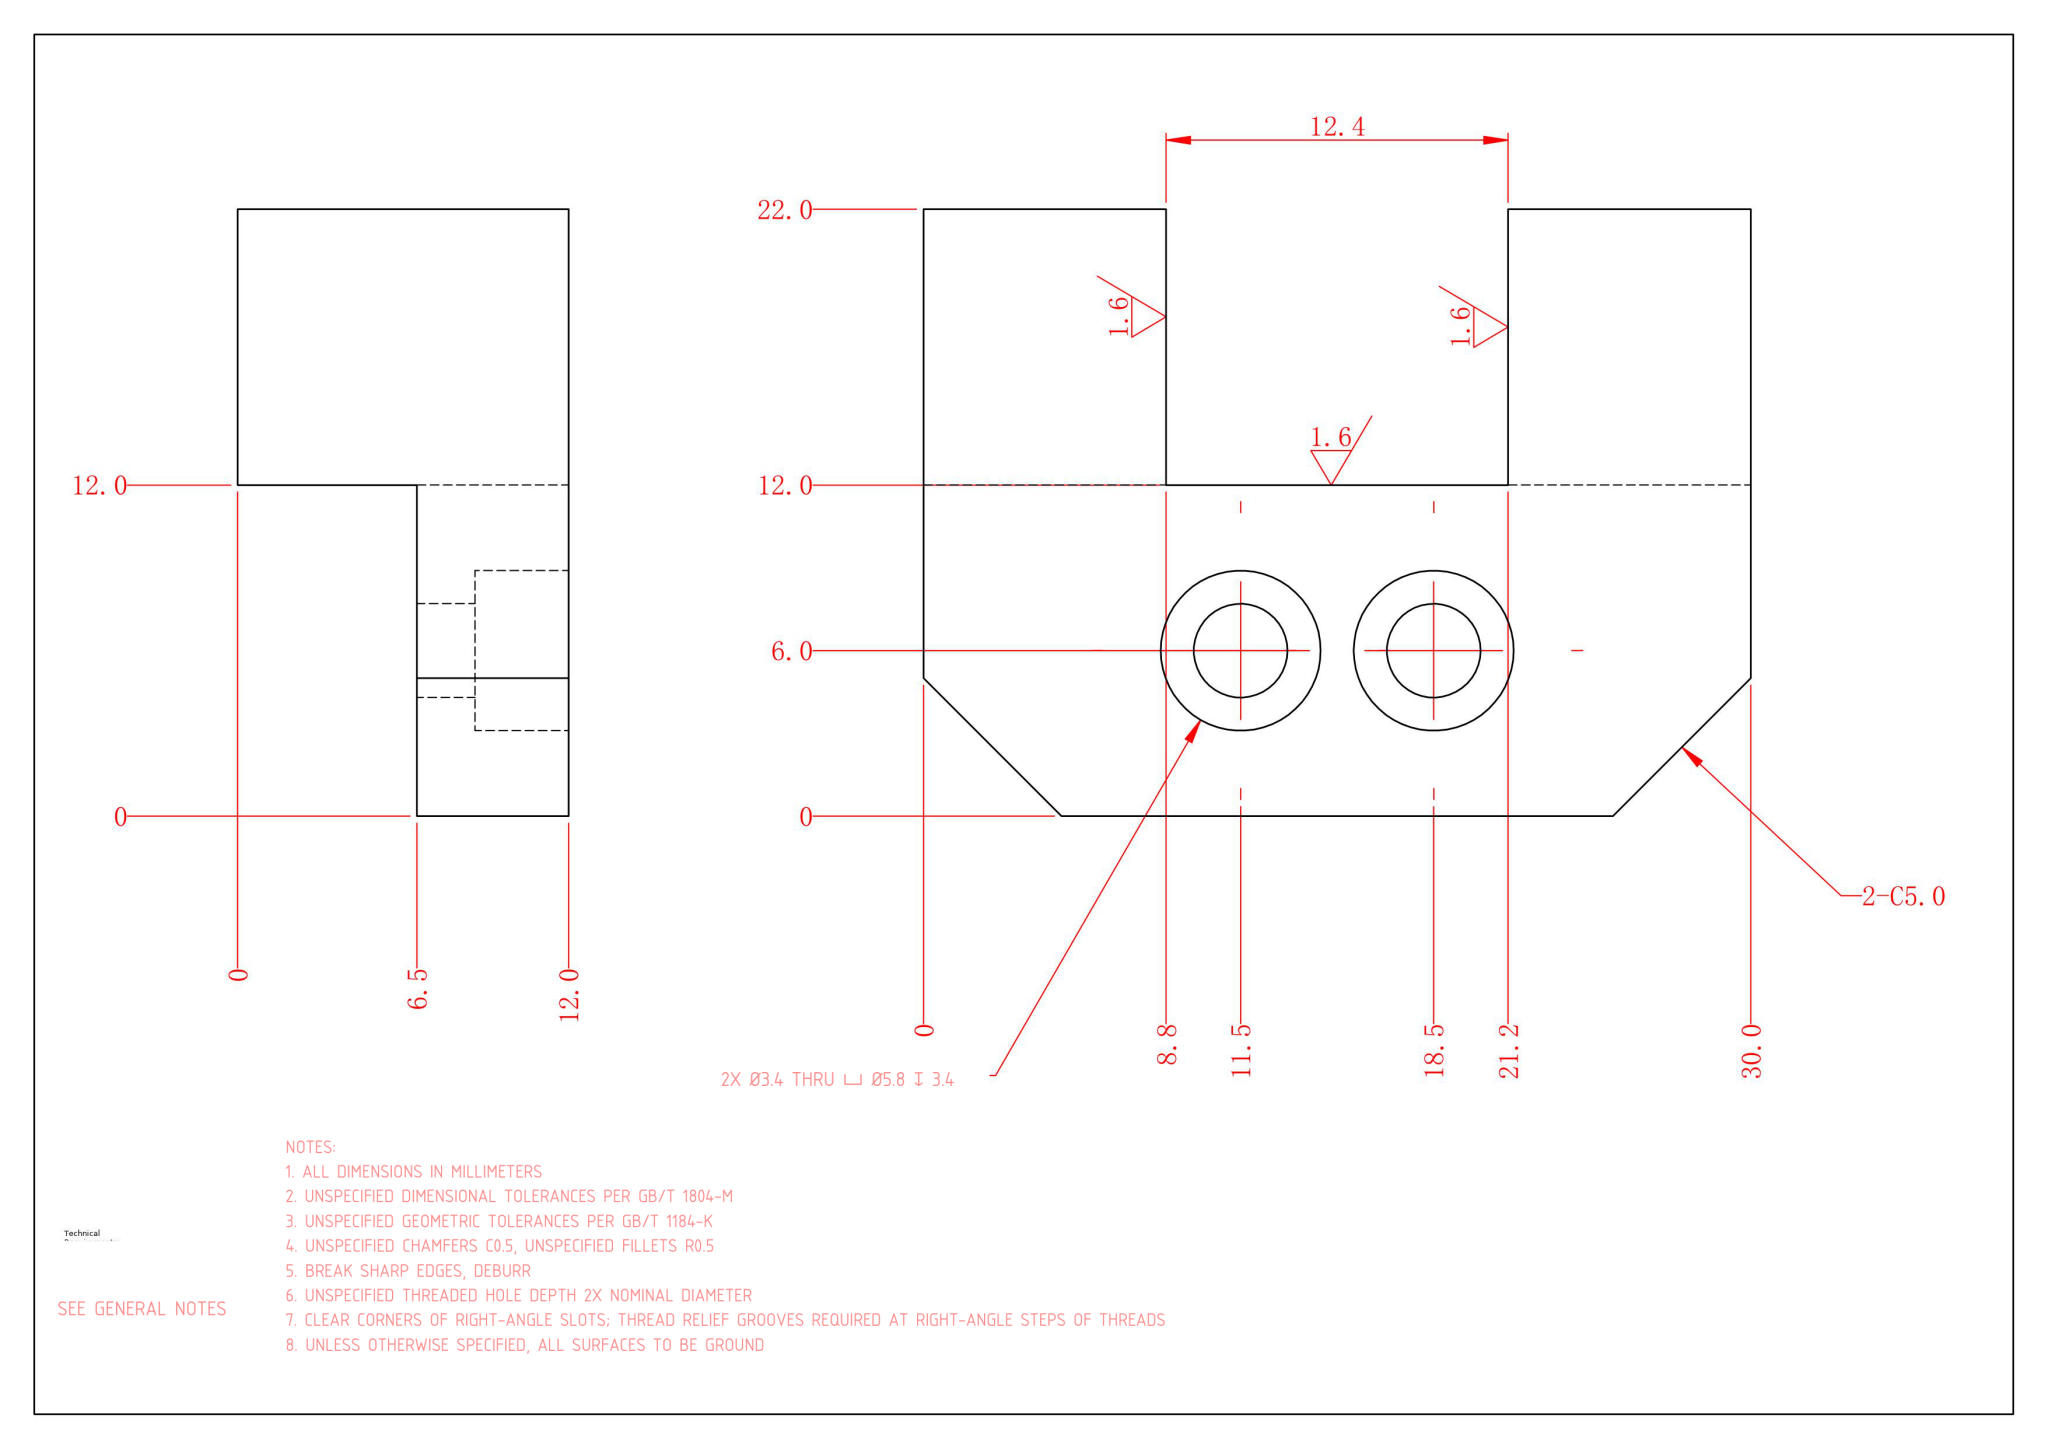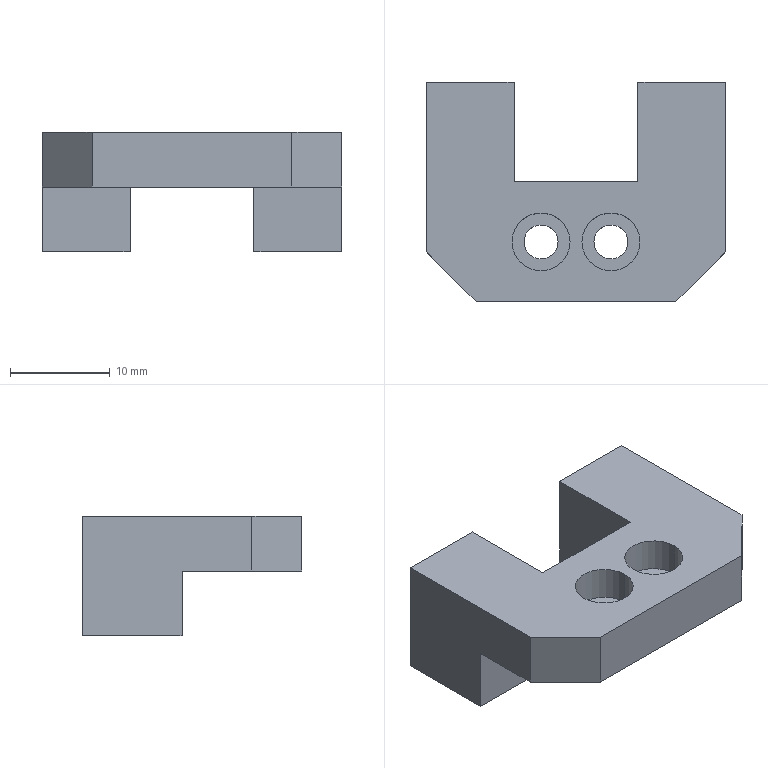Part | NX | mm | 1 solid | 26 faces | box 30 x 22 x 12 mm | volume 3737 mm3 | plane 18 | cylinder 8 | commonest cylinder face diameters 5.8 x4 3.4 x4
STEP:
#1=COLOUR_RGB('',0.7529,0.7529,0.7529);
#2=FILL_AREA_STYLE_COLOUR('',#1);
#3=FILL_AREA_STYLE('',(#2));
#4=SURFACE_STYLE_FILL_AREA(#3);
#5=SURFACE_SIDE_STYLE('',(#4));
#6=SURFACE_STYLE_USAGE(.BOTH.,#5);
#7=PRESENTATION_STYLE_ASSIGNMENT((#6));
#8=CARTESIAN_POINT('',(0.6,-5.,8.6));
#9=VERTEX_POINT('',#8);
#10=CARTESIAN_POINT('',(6.4,-5.,8.6));
#11=VERTEX_POINT('',#10);
#12=CARTESIAN_POINT('',(3.5,-5.,8.6));
#13=DIRECTION('',(0.,0.,1.));
#14=DIRECTION('',(1.,0.,0.));
#15=AXIS2_PLACEMENT_3D('',#12,#13,#14);
#16=CIRCLE('',#15,2.9);
#17=EDGE_CURVE('',#9,#11,#16,.T.);
#18=ORIENTED_EDGE('',*,*,#17,.F.);
#19=CARTESIAN_POINT('',(0.6,-5.,12.));
#20=VERTEX_POINT('',#19);
#21=CARTESIAN_POINT('',(0.6,-5.,12.));
#22=DIRECTION('',(0.,0.,1.));
#23=VECTOR('',#22,1000.);
#24=LINE('',#21,#23);
#25=EDGE_CURVE('',#9,#20,#24,.T.);
#26=ORIENTED_EDGE('',*,*,#25,.T.);
#27=CARTESIAN_POINT('',(6.4,-5.,12.));
#28=VERTEX_POINT('',#27);
#29=CARTESIAN_POINT('',(3.5,-5.,12.));
#30=DIRECTION('',(0.,0.,1.));
#31=DIRECTION('',(1.,0.,0.));
#32=AXIS2_PLACEMENT_3D('',#29,#30,#31);
#33=CIRCLE('',#32,2.9);
#34=EDGE_CURVE('',#20,#28,#33,.T.);
#35=ORIENTED_EDGE('',*,*,#34,.T.);
#36=CARTESIAN_POINT('',(6.4,-5.,12.));
#37=DIRECTION('',(0.,0.,1.));
#38=VECTOR('',#37,1000.);
#39=LINE('',#36,#38);
#40=EDGE_CURVE('',#11,#28,#39,.T.);
#41=ORIENTED_EDGE('',*,*,#40,.F.);
#42=EDGE_LOOP('',(#18,#26,#35,#41));
#43=FACE_OUTER_BOUND('',#42,.T.);
#44=CARTESIAN_POINT('',(3.5,-5.,12.));
#45=DIRECTION('',(0.,0.,1.));
#46=DIRECTION('',(1.,0.,0.));
#47=AXIS2_PLACEMENT_3D('',#44,#45,#46);
#48=CYLINDRICAL_SURFACE('',#47,2.9);
#49=ADVANCED_FACE('',(#43),#48,.F.);
#50=CARTESIAN_POINT('',(1.8,-5.,6.5));
#51=VERTEX_POINT('',#50);
#52=CARTESIAN_POINT('',(5.2,-5.,6.5));
#53=VERTEX_POINT('',#52);
#54=CARTESIAN_POINT('',(3.5,-5.,6.5));
#55=DIRECTION('',(0.,0.,1.));
#56=DIRECTION('',(1.,0.,0.));
#57=AXIS2_PLACEMENT_3D('',#54,#55,#56);
#58=CIRCLE('',#57,1.7);
#59=EDGE_CURVE('',#51,#53,#58,.T.);
#60=ORIENTED_EDGE('',*,*,#59,.F.);
#61=CARTESIAN_POINT('',(1.8,-5.,8.6));
#62=VERTEX_POINT('',#61);
#63=CARTESIAN_POINT('',(1.8,-5.,12.));
#64=DIRECTION('',(0.,0.,1.));
#65=VECTOR('',#64,1000.);
#66=LINE('',#63,#65);
#67=EDGE_CURVE('',#51,#62,#66,.T.);
#68=ORIENTED_EDGE('',*,*,#67,.T.);
#69=CARTESIAN_POINT('',(5.2,-5.,8.6));
#70=VERTEX_POINT('',#69);
#71=CARTESIAN_POINT('',(3.5,-5.,8.6));
#72=DIRECTION('',(0.,0.,1.));
#73=DIRECTION('',(1.,0.,0.));
#74=AXIS2_PLACEMENT_3D('',#71,#72,#73);
#75=CIRCLE('',#74,1.7);
#76=EDGE_CURVE('',#62,#70,#75,.T.);
#77=ORIENTED_EDGE('',*,*,#76,.T.);
#78=CARTESIAN_POINT('',(5.2,-5.,12.));
#79=DIRECTION('',(0.,0.,1.));
#80=VECTOR('',#79,1000.);
#81=LINE('',#78,#80);
#82=EDGE_CURVE('',#53,#70,#81,.T.);
#83=ORIENTED_EDGE('',*,*,#82,.F.);
#84=EDGE_LOOP('',(#60,#68,#77,#83));
#85=FACE_OUTER_BOUND('',#84,.T.);
#86=CARTESIAN_POINT('',(3.5,-5.,12.));
#87=DIRECTION('',(0.,0.,1.));
#88=DIRECTION('',(1.,0.,0.));
#89=AXIS2_PLACEMENT_3D('',#86,#87,#88);
#90=CYLINDRICAL_SURFACE('',#89,1.7);
#91=ADVANCED_FACE('',(#85),#90,.F.);
#92=CARTESIAN_POINT('',(-6.4,-5.,8.6));
#93=VERTEX_POINT('',#92);
#94=CARTESIAN_POINT('',(-0.6,-5.,8.6));
#95=VERTEX_POINT('',#94);
#96=CARTESIAN_POINT('',(-3.5,-5.,8.6));
#97=DIRECTION('',(0.,0.,1.));
#98=DIRECTION('',(1.,0.,0.));
#99=AXIS2_PLACEMENT_3D('',#96,#97,#98);
#100=CIRCLE('',#99,2.9);
#101=EDGE_CURVE('',#93,#95,#100,.T.);
#102=ORIENTED_EDGE('',*,*,#101,.F.);
#103=CARTESIAN_POINT('',(-6.4,-5.,12.));
#104=VERTEX_POINT('',#103);
#105=CARTESIAN_POINT('',(-6.4,-5.,12.));
#106=DIRECTION('',(0.,0.,1.));
#107=VECTOR('',#106,1000.);
#108=LINE('',#105,#107);
#109=EDGE_CURVE('',#93,#104,#108,.T.);
#110=ORIENTED_EDGE('',*,*,#109,.T.);
#111=CARTESIAN_POINT('',(-0.6,-5.,12.));
#112=VERTEX_POINT('',#111);
#113=CARTESIAN_POINT('',(-3.5,-5.,12.));
#114=DIRECTION('',(0.,0.,1.));
#115=DIRECTION('',(1.,0.,0.));
#116=AXIS2_PLACEMENT_3D('',#113,#114,#115);
#117=CIRCLE('',#116,2.9);
#118=EDGE_CURVE('',#104,#112,#117,.T.);
#119=ORIENTED_EDGE('',*,*,#118,.T.);
#120=CARTESIAN_POINT('',(-0.6,-5.,12.));
#121=DIRECTION('',(0.,0.,1.));
#122=VECTOR('',#121,1000.);
#123=LINE('',#120,#122);
#124=EDGE_CURVE('',#95,#112,#123,.T.);
#125=ORIENTED_EDGE('',*,*,#124,.F.);
#126=EDGE_LOOP('',(#102,#110,#119,#125));
#127=FACE_OUTER_BOUND('',#126,.T.);
#128=CARTESIAN_POINT('',(-3.5,-5.,12.));
#129=DIRECTION('',(0.,0.,1.));
#130=DIRECTION('',(1.,0.,0.));
#131=AXIS2_PLACEMENT_3D('',#128,#129,#130);
#132=CYLINDRICAL_SURFACE('',#131,2.9);
#133=ADVANCED_FACE('',(#127),#132,.F.);
#134=CARTESIAN_POINT('',(-5.2,-5.,6.5));
#135=VERTEX_POINT('',#134);
#136=CARTESIAN_POINT('',(-1.8,-5.,6.5));
#137=VERTEX_POINT('',#136);
#138=CARTESIAN_POINT('',(-3.5,-5.,6.5));
#139=DIRECTION('',(0.,0.,1.));
#140=DIRECTION('',(1.,0.,0.));
#141=AXIS2_PLACEMENT_3D('',#138,#139,#140);
#142=CIRCLE('',#141,1.7);
#143=EDGE_CURVE('',#135,#137,#142,.T.);
#144=ORIENTED_EDGE('',*,*,#143,.F.);
#145=CARTESIAN_POINT('',(-5.2,-5.,8.6));
#146=VERTEX_POINT('',#145);
#147=CARTESIAN_POINT('',(-5.2,-5.,12.));
#148=DIRECTION('',(0.,0.,1.));
#149=VECTOR('',#148,1000.);
#150=LINE('',#147,#149);
#151=EDGE_CURVE('',#135,#146,#150,.T.);
#152=ORIENTED_EDGE('',*,*,#151,.T.);
#153=CARTESIAN_POINT('',(-1.8,-5.,8.6));
#154=VERTEX_POINT('',#153);
#155=CARTESIAN_POINT('',(-3.5,-5.,8.6));
#156=DIRECTION('',(0.,0.,1.));
#157=DIRECTION('',(1.,0.,0.));
#158=AXIS2_PLACEMENT_3D('',#155,#156,#157);
#159=CIRCLE('',#158,1.7);
#160=EDGE_CURVE('',#146,#154,#159,.T.);
#161=ORIENTED_EDGE('',*,*,#160,.T.);
#162=CARTESIAN_POINT('',(-1.8,-5.,12.));
#163=DIRECTION('',(0.,0.,1.));
#164=VECTOR('',#163,1000.);
#165=LINE('',#162,#164);
#166=EDGE_CURVE('',#137,#154,#165,.T.);
#167=ORIENTED_EDGE('',*,*,#166,.F.);
#168=EDGE_LOOP('',(#144,#152,#161,#167));
#169=FACE_OUTER_BOUND('',#168,.T.);
#170=CARTESIAN_POINT('',(-3.5,-5.,12.));
#171=DIRECTION('',(0.,0.,1.));
#172=DIRECTION('',(1.,0.,0.));
#173=AXIS2_PLACEMENT_3D('',#170,#171,#172);
#174=CYLINDRICAL_SURFACE('',#173,1.7);
#175=ADVANCED_FACE('',(#169),#174,.F.);
#176=CARTESIAN_POINT('',(15.,1.,0.));
#177=VERTEX_POINT('',#176);
#178=CARTESIAN_POINT('',(15.,11.,0.));
#179=VERTEX_POINT('',#178);
#180=CARTESIAN_POINT('',(15.,11.,0.));
#181=DIRECTION('',(-0.,1.,0.));
#182=VECTOR('',#181,1000.);
#183=LINE('',#180,#182);
#184=EDGE_CURVE('',#177,#179,#183,.T.);
#185=ORIENTED_EDGE('',*,*,#184,.F.);
#186=CARTESIAN_POINT('',(6.2,1.,0.));
#187=VERTEX_POINT('',#186);
#188=CARTESIAN_POINT('',(15.001,1.,0.));
#189=DIRECTION('',(-1.,-0.,0.));
#190=VECTOR('',#189,1000.);
#191=LINE('',#188,#190);
#192=EDGE_CURVE('',#177,#187,#191,.T.);
#193=ORIENTED_EDGE('',*,*,#192,.T.);
#194=CARTESIAN_POINT('',(6.2,11.,0.));
#195=VERTEX_POINT('',#194);
#196=CARTESIAN_POINT('',(6.2,11.,0.));
#197=DIRECTION('',(0.,-1.,0.));
#198=VECTOR('',#197,1000.);
#199=LINE('',#196,#198);
#200=EDGE_CURVE('',#195,#187,#199,.T.);
#201=ORIENTED_EDGE('',*,*,#200,.F.);
#202=CARTESIAN_POINT('',(-15.,11.,0.));
#203=DIRECTION('',(-1.,0.,0.));
#204=VECTOR('',#203,1000.);
#205=LINE('',#202,#204);
#206=EDGE_CURVE('',#179,#195,#205,.T.);
#207=ORIENTED_EDGE('',*,*,#206,.F.);
#208=EDGE_LOOP('',(#185,#193,#201,#207));
#209=FACE_OUTER_BOUND('',#208,.T.);
#210=CARTESIAN_POINT('',(0.,0.,0.));
#211=DIRECTION('',(0.,0.,1.));
#212=DIRECTION('',(1.,0.,0.));
#213=AXIS2_PLACEMENT_3D('',#210,#211,#212);
#214=PLANE('',#213);
#215=ADVANCED_FACE('',(#209),#214,.F.);
#216=CARTESIAN_POINT('',(-6.2,11.,12.));
#217=VERTEX_POINT('',#216);
#218=CARTESIAN_POINT('',(-15.,11.,12.));
#219=VERTEX_POINT('',#218);
#220=CARTESIAN_POINT('',(-15.,11.,12.));
#221=DIRECTION('',(-1.,0.,0.));
#222=VECTOR('',#221,1000.);
#223=LINE('',#220,#222);
#224=EDGE_CURVE('',#217,#219,#223,.T.);
#225=ORIENTED_EDGE('',*,*,#224,.F.);
#226=CARTESIAN_POINT('',(-6.2,11.,0.));
#227=VERTEX_POINT('',#226);
#228=CARTESIAN_POINT('',(-6.2,11.,-0.001));
#229=DIRECTION('',(0.,0.,1.));
#230=VECTOR('',#229,1000.);
#231=LINE('',#228,#230);
#232=EDGE_CURVE('',#227,#217,#231,.T.);
#233=ORIENTED_EDGE('',*,*,#232,.F.);
#234=CARTESIAN_POINT('',(-15.,11.,0.));
#235=VERTEX_POINT('',#234);
#236=CARTESIAN_POINT('',(-15.,11.,0.));
#237=DIRECTION('',(-1.,0.,0.));
#238=VECTOR('',#237,1000.);
#239=LINE('',#236,#238);
#240=EDGE_CURVE('',#227,#235,#239,.T.);
#241=ORIENTED_EDGE('',*,*,#240,.T.);
#242=CARTESIAN_POINT('',(-15.,11.,12.));
#243=DIRECTION('',(0.,0.,-1.));
#244=VECTOR('',#243,1000.);
#245=LINE('',#242,#244);
#246=EDGE_CURVE('',#219,#235,#245,.T.);
#247=ORIENTED_EDGE('',*,*,#246,.F.);
#248=EDGE_LOOP('',(#225,#233,#241,#247));
#249=FACE_OUTER_BOUND('',#248,.T.);
#250=CARTESIAN_POINT('',(-15.,11.,12.));
#251=DIRECTION('',(0.,-1.,0.));
#252=DIRECTION('',(0.,0.,-1.));
#253=AXIS2_PLACEMENT_3D('',#250,#251,#252);
#254=PLANE('',#253);
#255=ADVANCED_FACE('',(#249),#254,.F.);
#256=CARTESIAN_POINT('',(15.,-6.,12.));
#257=VERTEX_POINT('',#256);
#258=CARTESIAN_POINT('',(15.,11.,12.));
#259=VERTEX_POINT('',#258);
#260=CARTESIAN_POINT('',(15.,11.,12.));
#261=DIRECTION('',(-0.,1.,0.));
#262=VECTOR('',#261,1000.);
#263=LINE('',#260,#262);
#264=EDGE_CURVE('',#257,#259,#263,.T.);
#265=ORIENTED_EDGE('',*,*,#264,.F.);
#266=CARTESIAN_POINT('',(15.,-6.,6.5));
#267=VERTEX_POINT('',#266);
#268=CARTESIAN_POINT('',(15.,-6.,12.));
#269=DIRECTION('',(0.,0.,-1.));
#270=VECTOR('',#269,1000.);
#271=LINE('',#268,#270);
#272=EDGE_CURVE('',#257,#267,#271,.T.);
#273=ORIENTED_EDGE('',*,*,#272,.T.);
#274=CARTESIAN_POINT('',(15.,1.,6.5));
#275=VERTEX_POINT('',#274);
#276=CARTESIAN_POINT('',(15.,-11.,6.5));
#277=DIRECTION('',(0.,-1.,0.));
#278=VECTOR('',#277,1000.);
#279=LINE('',#276,#278);
#280=EDGE_CURVE('',#275,#267,#279,.T.);
#281=ORIENTED_EDGE('',*,*,#280,.F.);
#282=CARTESIAN_POINT('',(15.,1.,0.));
#283=DIRECTION('',(0.,0.,1.));
#284=VECTOR('',#283,1000.);
#285=LINE('',#282,#284);
#286=EDGE_CURVE('',#177,#275,#285,.T.);
#287=ORIENTED_EDGE('',*,*,#286,.F.);
#288=ORIENTED_EDGE('',*,*,#184,.T.);
#289=CARTESIAN_POINT('',(15.,11.,12.));
#290=DIRECTION('',(0.,0.,-1.));
#291=VECTOR('',#290,1000.);
#292=LINE('',#289,#291);
#293=EDGE_CURVE('',#259,#179,#292,.T.);
#294=ORIENTED_EDGE('',*,*,#293,.F.);
#295=EDGE_LOOP('',(#265,#273,#281,#287,#288,#294));
#296=FACE_OUTER_BOUND('',#295,.T.);
#297=CARTESIAN_POINT('',(15.,11.,12.));
#298=DIRECTION('',(-1.,-0.,0.));
#299=DIRECTION('',(0.,-1.,0.));
#300=AXIS2_PLACEMENT_3D('',#297,#298,#299);
#301=PLANE('',#300);
#302=ADVANCED_FACE('',(#296),#301,.F.);
#303=ORIENTED_EDGE('',*,*,#206,.T.);
#304=CARTESIAN_POINT('',(6.2,11.,12.));
#305=VERTEX_POINT('',#304);
#306=CARTESIAN_POINT('',(6.2,11.,-0.001));
#307=DIRECTION('',(0.,0.,1.));
#308=VECTOR('',#307,1000.);
#309=LINE('',#306,#308);
#310=EDGE_CURVE('',#195,#305,#309,.T.);
#311=ORIENTED_EDGE('',*,*,#310,.T.);
#312=CARTESIAN_POINT('',(-15.,11.,12.));
#313=DIRECTION('',(-1.,0.,0.));
#314=VECTOR('',#313,1000.);
#315=LINE('',#312,#314);
#316=EDGE_CURVE('',#259,#305,#315,.T.);
#317=ORIENTED_EDGE('',*,*,#316,.F.);
#318=ORIENTED_EDGE('',*,*,#293,.T.);
#319=EDGE_LOOP('',(#303,#311,#317,#318));
#320=FACE_OUTER_BOUND('',#319,.T.);
#321=CARTESIAN_POINT('',(-15.,11.,12.));
#322=DIRECTION('',(0.,-1.,0.));
#323=DIRECTION('',(0.,0.,-1.));
#324=AXIS2_PLACEMENT_3D('',#321,#322,#323);
#325=PLANE('',#324);
#326=ADVANCED_FACE('',(#320),#325,.F.);
#327=CARTESIAN_POINT('',(-15.,-6.,6.5));
#328=VERTEX_POINT('',#327);
#329=CARTESIAN_POINT('',(-15.,1.,6.5));
#330=VERTEX_POINT('',#329);
#331=CARTESIAN_POINT('',(-15.,-11.,6.5));
#332=DIRECTION('',(-0.,1.,0.));
#333=VECTOR('',#332,1000.);
#334=LINE('',#331,#333);
#335=EDGE_CURVE('',#328,#330,#334,.T.);
#336=ORIENTED_EDGE('',*,*,#335,.F.);
#337=CARTESIAN_POINT('',(-15.,-6.,12.));
#338=VERTEX_POINT('',#337);
#339=CARTESIAN_POINT('',(-15.,-6.,12.));
#340=DIRECTION('',(0.,0.,1.));
#341=VECTOR('',#340,1000.);
#342=LINE('',#339,#341);
#343=EDGE_CURVE('',#328,#338,#342,.T.);
#344=ORIENTED_EDGE('',*,*,#343,.T.);
#345=CARTESIAN_POINT('',(-15.,11.,12.));
#346=DIRECTION('',(0.,-1.,0.));
#347=VECTOR('',#346,1000.);
#348=LINE('',#345,#347);
#349=EDGE_CURVE('',#219,#338,#348,.T.);
#350=ORIENTED_EDGE('',*,*,#349,.F.);
#351=ORIENTED_EDGE('',*,*,#246,.T.);
#352=CARTESIAN_POINT('',(-15.,1.,0.));
#353=VERTEX_POINT('',#352);
#354=CARTESIAN_POINT('',(-15.,11.,0.));
#355=DIRECTION('',(0.,-1.,0.));
#356=VECTOR('',#355,1000.);
#357=LINE('',#354,#356);
#358=EDGE_CURVE('',#235,#353,#357,.T.);
#359=ORIENTED_EDGE('',*,*,#358,.T.);
#360=CARTESIAN_POINT('',(-15.,1.,0.));
#361=DIRECTION('',(0.,0.,-1.));
#362=VECTOR('',#361,1000.);
#363=LINE('',#360,#362);
#364=EDGE_CURVE('',#330,#353,#363,.T.);
#365=ORIENTED_EDGE('',*,*,#364,.F.);
#366=EDGE_LOOP('',(#336,#344,#350,#351,#359,#365));
#367=FACE_OUTER_BOUND('',#366,.T.);
#368=CARTESIAN_POINT('',(-15.,11.,12.));
#369=DIRECTION('',(1.,0.,0.));
#370=DIRECTION('',(-0.,1.,0.));
#371=AXIS2_PLACEMENT_3D('',#368,#369,#370);
#372=PLANE('',#371);
#373=ADVANCED_FACE('',(#367),#372,.F.);
#374=CARTESIAN_POINT('',(10.,-11.,6.5));
#375=VERTEX_POINT('',#374);
#376=CARTESIAN_POINT('',(-10.,-11.,6.5));
#377=VERTEX_POINT('',#376);
#378=CARTESIAN_POINT('',(15.001,-11.,6.5));
#379=DIRECTION('',(-1.,-0.,0.));
#380=VECTOR('',#379,1000.);
#381=LINE('',#378,#380);
#382=EDGE_CURVE('',#375,#377,#381,.T.);
#383=ORIENTED_EDGE('',*,*,#382,.F.);
#384=CARTESIAN_POINT('',(10.,-11.,12.));
#385=VERTEX_POINT('',#384);
#386=CARTESIAN_POINT('',(10.,-11.,12.));
#387=DIRECTION('',(0.,0.,1.));
#388=VECTOR('',#387,1000.);
#389=LINE('',#386,#388);
#390=EDGE_CURVE('',#375,#385,#389,.T.);
#391=ORIENTED_EDGE('',*,*,#390,.T.);
#392=CARTESIAN_POINT('',(-10.,-11.,12.));
#393=VERTEX_POINT('',#392);
#394=CARTESIAN_POINT('',(-15.,-11.,12.));
#395=DIRECTION('',(1.,0.,0.));
#396=VECTOR('',#395,1000.);
#397=LINE('',#394,#396);
#398=EDGE_CURVE('',#393,#385,#397,.T.);
#399=ORIENTED_EDGE('',*,*,#398,.F.);
#400=CARTESIAN_POINT('',(-10.,-11.,12.));
#401=DIRECTION('',(0.,0.,-1.));
#402=VECTOR('',#401,1000.);
#403=LINE('',#400,#402);
#404=EDGE_CURVE('',#393,#377,#403,.T.);
#405=ORIENTED_EDGE('',*,*,#404,.T.);
#406=EDGE_LOOP('',(#383,#391,#399,#405));
#407=FACE_OUTER_BOUND('',#406,.T.);
#408=CARTESIAN_POINT('',(-15.,-11.,12.));
#409=DIRECTION('',(0.,1.,0.));
#410=DIRECTION('',(0.,0.,1.));
#411=AXIS2_PLACEMENT_3D('',#408,#409,#410);
#412=PLANE('',#411);
#413=ADVANCED_FACE('',(#407),#412,.F.);
#414=CARTESIAN_POINT('',(3.5,-5.,12.));
#415=DIRECTION('',(0.,0.,1.));
#416=DIRECTION('',(1.,0.,0.));
#417=AXIS2_PLACEMENT_3D('',#414,#415,#416);
#418=CIRCLE('',#417,2.9);
#419=EDGE_CURVE('',#28,#20,#418,.T.);
#420=ORIENTED_EDGE('',*,*,#419,.F.);
#421=ORIENTED_EDGE('',*,*,#34,.F.);
#422=EDGE_LOOP('',(#420,#421));
#423=FACE_BOUND('',#422,.T.);
#424=CARTESIAN_POINT('',(-3.5,-5.,12.));
#425=DIRECTION('',(0.,0.,1.));
#426=DIRECTION('',(1.,0.,0.));
#427=AXIS2_PLACEMENT_3D('',#424,#425,#426);
#428=CIRCLE('',#427,2.9);
#429=EDGE_CURVE('',#112,#104,#428,.T.);
#430=ORIENTED_EDGE('',*,*,#429,.F.);
#431=ORIENTED_EDGE('',*,*,#118,.F.);
#432=EDGE_LOOP('',(#430,#431));
#433=FACE_BOUND('',#432,.T.);
#434=ORIENTED_EDGE('',*,*,#398,.T.);
#435=CARTESIAN_POINT('',(10.5,-10.5,12.));
#436=DIRECTION('',(0.7071,0.7071,0.));
#437=VECTOR('',#436,1000.);
#438=LINE('',#435,#437);
#439=EDGE_CURVE('',#385,#257,#438,.T.);
#440=ORIENTED_EDGE('',*,*,#439,.T.);
#441=ORIENTED_EDGE('',*,*,#264,.T.);
#442=ORIENTED_EDGE('',*,*,#316,.T.);
#443=CARTESIAN_POINT('',(6.2,1.,12.));
#444=VERTEX_POINT('',#443);
#445=CARTESIAN_POINT('',(6.2,11.,12.));
#446=DIRECTION('',(-0.,1.,0.));
#447=VECTOR('',#446,1000.);
#448=LINE('',#445,#447);
#449=EDGE_CURVE('',#444,#305,#448,.T.);
#450=ORIENTED_EDGE('',*,*,#449,.F.);
#451=CARTESIAN_POINT('',(-6.2,1.,12.));
#452=VERTEX_POINT('',#451);
#453=CARTESIAN_POINT('',(-6.2,1.,12.));
#454=DIRECTION('',(1.,0.,0.));
#455=VECTOR('',#454,1000.);
#456=LINE('',#453,#455);
#457=EDGE_CURVE('',#452,#444,#456,.T.);
#458=ORIENTED_EDGE('',*,*,#457,.F.);
#459=CARTESIAN_POINT('',(-6.2,11.,12.));
#460=DIRECTION('',(-0.,-1.,0.));
#461=VECTOR('',#460,1000.);
#462=LINE('',#459,#461);
#463=EDGE_CURVE('',#217,#452,#462,.T.);
#464=ORIENTED_EDGE('',*,*,#463,.F.);
#465=ORIENTED_EDGE('',*,*,#224,.T.);
#466=ORIENTED_EDGE('',*,*,#349,.T.);
#467=CARTESIAN_POINT('',(-10.5,-10.5,12.));
#468=DIRECTION('',(0.7071,-0.7071,0.));
#469=VECTOR('',#468,1000.);
#470=LINE('',#467,#469);
#471=EDGE_CURVE('',#338,#393,#470,.T.);
#472=ORIENTED_EDGE('',*,*,#471,.T.);
#473=EDGE_LOOP('',(#434,#440,#441,#442,#450,#458,#464,#465,#466,#472));
#474=FACE_OUTER_BOUND('',#473,.T.);
#475=CARTESIAN_POINT('',(0.,0.,12.));
#476=DIRECTION('',(0.,0.,1.));
#477=DIRECTION('',(1.,0.,0.));
#478=AXIS2_PLACEMENT_3D('',#475,#476,#477);
#479=PLANE('',#478);
#480=ADVANCED_FACE('',(#423,#433,#474),#479,.T.);
#481=CARTESIAN_POINT('',(-6.2,1.,0.));
#482=VERTEX_POINT('',#481);
#483=CARTESIAN_POINT('',(-6.2,11.,0.));
#484=DIRECTION('',(0.,1.,0.));
#485=VECTOR('',#484,1000.);
#486=LINE('',#483,#485);
#487=EDGE_CURVE('',#482,#227,#486,.T.);
#488=ORIENTED_EDGE('',*,*,#487,.F.);
#489=CARTESIAN_POINT('',(15.001,1.,0.));
#490=DIRECTION('',(-1.,-0.,0.));
#491=VECTOR('',#490,1000.);
#492=LINE('',#489,#491);
#493=EDGE_CURVE('',#482,#353,#492,.T.);
#494=ORIENTED_EDGE('',*,*,#493,.T.);
#495=ORIENTED_EDGE('',*,*,#358,.F.);
#496=ORIENTED_EDGE('',*,*,#240,.F.);
#497=EDGE_LOOP('',(#488,#494,#495,#496));
#498=FACE_OUTER_BOUND('',#497,.T.);
#499=CARTESIAN_POINT('',(0.,0.,0.));
#500=DIRECTION('',(0.,0.,1.));
#501=DIRECTION('',(1.,0.,0.));
#502=AXIS2_PLACEMENT_3D('',#499,#500,#501);
#503=PLANE('',#502);
#504=ADVANCED_FACE('',(#498),#503,.F.);
#505=ORIENTED_EDGE('',*,*,#487,.T.);
#506=ORIENTED_EDGE('',*,*,#232,.T.);
#507=ORIENTED_EDGE('',*,*,#463,.T.);
#508=CARTESIAN_POINT('',(-6.2,1.,6.5));
#509=VERTEX_POINT('',#508);
#510=CARTESIAN_POINT('',(-6.2,1.,-0.001));
#511=DIRECTION('',(0.,0.,1.));
#512=VECTOR('',#511,1000.);
#513=LINE('',#510,#512);
#514=EDGE_CURVE('',#509,#452,#513,.T.);
#515=ORIENTED_EDGE('',*,*,#514,.F.);
#516=CARTESIAN_POINT('',(-6.2,1.,-0.001));
#517=DIRECTION('',(0.,0.,1.));
#518=VECTOR('',#517,1000.);
#519=LINE('',#516,#518);
#520=EDGE_CURVE('',#482,#509,#519,.T.);
#521=ORIENTED_EDGE('',*,*,#520,.F.);
#522=EDGE_LOOP('',(#505,#506,#507,#515,#521));
#523=FACE_OUTER_BOUND('',#522,.T.);
#524=CARTESIAN_POINT('',(-6.2,11.,-0.001));
#525=DIRECTION('',(-1.,0.,0.));
#526=DIRECTION('',(-0.,-1.,0.));
#527=AXIS2_PLACEMENT_3D('',#524,#525,#526);
#528=PLANE('',#527);
#529=ADVANCED_FACE('',(#523),#528,.F.);
#530=ORIENTED_EDGE('',*,*,#200,.T.);
#531=CARTESIAN_POINT('',(6.2,1.,6.5));
#532=VERTEX_POINT('',#531);
#533=CARTESIAN_POINT('',(6.2,1.,-0.001));
#534=DIRECTION('',(0.,0.,1.));
#535=VECTOR('',#534,1000.);
#536=LINE('',#533,#535);
#537=EDGE_CURVE('',#187,#532,#536,.T.);
#538=ORIENTED_EDGE('',*,*,#537,.T.);
#539=CARTESIAN_POINT('',(6.2,1.,-0.001));
#540=DIRECTION('',(0.,0.,1.));
#541=VECTOR('',#540,1000.);
#542=LINE('',#539,#541);
#543=EDGE_CURVE('',#532,#444,#542,.T.);
#544=ORIENTED_EDGE('',*,*,#543,.T.);
#545=ORIENTED_EDGE('',*,*,#449,.T.);
#546=ORIENTED_EDGE('',*,*,#310,.F.);
#547=EDGE_LOOP('',(#530,#538,#544,#545,#546));
#548=FACE_OUTER_BOUND('',#547,.T.);
#549=CARTESIAN_POINT('',(6.2,11.,-0.001));
#550=DIRECTION('',(1.,0.,0.));
#551=DIRECTION('',(-0.,1.,0.));
#552=AXIS2_PLACEMENT_3D('',#549,#550,#551);
#553=PLANE('',#552);
#554=ADVANCED_FACE('',(#548),#553,.F.);
#555=ORIENTED_EDGE('',*,*,#543,.F.);
#556=CARTESIAN_POINT('',(-6.2,1.,6.5));
#557=DIRECTION('',(-1.,0.,0.));
#558=VECTOR('',#557,1000.);
#559=LINE('',#556,#558);
#560=EDGE_CURVE('',#532,#509,#559,.T.);
#561=ORIENTED_EDGE('',*,*,#560,.T.);
#562=ORIENTED_EDGE('',*,*,#514,.T.);
#563=ORIENTED_EDGE('',*,*,#457,.T.);
#564=EDGE_LOOP('',(#555,#561,#562,#563));
#565=FACE_OUTER_BOUND('',#564,.T.);
#566=CARTESIAN_POINT('',(-6.2,1.,-0.001));
#567=DIRECTION('',(0.,-1.,0.));
#568=DIRECTION('',(0.,0.,-1.));
#569=AXIS2_PLACEMENT_3D('',#566,#567,#568);
#570=PLANE('',#569);
#571=ADVANCED_FACE('',(#565),#570,.F.);
#572=CARTESIAN_POINT('',(15.001,1.,6.5));
#573=DIRECTION('',(-1.,-0.,0.));
#574=VECTOR('',#573,1000.);
#575=LINE('',#572,#574);
#576=EDGE_CURVE('',#509,#330,#575,.T.);
#577=ORIENTED_EDGE('',*,*,#576,.T.);
#578=ORIENTED_EDGE('',*,*,#364,.T.);
#579=ORIENTED_EDGE('',*,*,#493,.F.);
#580=ORIENTED_EDGE('',*,*,#520,.T.);
#581=EDGE_LOOP('',(#577,#578,#579,#580));
#582=FACE_OUTER_BOUND('',#581,.T.);
#583=CARTESIAN_POINT('',(15.001,1.,0.));
#584=DIRECTION('',(-0.,1.,0.));
#585=DIRECTION('',(-1.,-0.,0.));
#586=AXIS2_PLACEMENT_3D('',#583,#584,#585);
#587=PLANE('',#586);
#588=ADVANCED_FACE('',(#582),#587,.F.);
#589=ORIENTED_EDGE('',*,*,#192,.F.);
#590=ORIENTED_EDGE('',*,*,#286,.T.);
#591=CARTESIAN_POINT('',(15.001,1.,6.5));
#592=DIRECTION('',(-1.,-0.,0.));
#593=VECTOR('',#592,1000.);
#594=LINE('',#591,#593);
#595=EDGE_CURVE('',#275,#532,#594,.T.);
#596=ORIENTED_EDGE('',*,*,#595,.T.);
#597=ORIENTED_EDGE('',*,*,#537,.F.);
#598=EDGE_LOOP('',(#589,#590,#596,#597));
#599=FACE_OUTER_BOUND('',#598,.T.);
#600=CARTESIAN_POINT('',(15.001,1.,0.));
#601=DIRECTION('',(-0.,1.,0.));
#602=DIRECTION('',(-1.,-0.,0.));
#603=AXIS2_PLACEMENT_3D('',#600,#601,#602);
#604=PLANE('',#603);
#605=ADVANCED_FACE('',(#599),#604,.F.);
#606=CARTESIAN_POINT('',(3.5,-5.,6.5));
#607=DIRECTION('',(0.,0.,1.));
#608=DIRECTION('',(1.,0.,0.));
#609=AXIS2_PLACEMENT_3D('',#606,#607,#608);
#610=CIRCLE('',#609,1.7);
#611=EDGE_CURVE('',#53,#51,#610,.T.);
#612=ORIENTED_EDGE('',*,*,#611,.T.);
#613=ORIENTED_EDGE('',*,*,#59,.T.);
#614=EDGE_LOOP('',(#612,#613));
#615=FACE_BOUND('',#614,.T.);
#616=CARTESIAN_POINT('',(-3.5,-5.,6.5));
#617=DIRECTION('',(0.,0.,1.));
#618=DIRECTION('',(1.,0.,0.));
#619=AXIS2_PLACEMENT_3D('',#616,#617,#618);
#620=CIRCLE('',#619,1.7);
#621=EDGE_CURVE('',#137,#135,#620,.T.);
#622=ORIENTED_EDGE('',*,*,#621,.T.);
#623=ORIENTED_EDGE('',*,*,#143,.T.);
#624=EDGE_LOOP('',(#622,#623));
#625=FACE_BOUND('',#624,.T.);
#626=ORIENTED_EDGE('',*,*,#280,.T.);
#627=CARTESIAN_POINT('',(15.,-6.,6.5));
#628=DIRECTION('',(-0.7071,-0.7071,0.));
#629=VECTOR('',#628,1000.);
#630=LINE('',#627,#629);
#631=EDGE_CURVE('',#267,#375,#630,.T.);
#632=ORIENTED_EDGE('',*,*,#631,.T.);
#633=ORIENTED_EDGE('',*,*,#382,.T.);
#634=CARTESIAN_POINT('',(-10.,-11.,6.5));
#635=DIRECTION('',(-0.7071,0.7071,0.));
#636=VECTOR('',#635,1000.);
#637=LINE('',#634,#636);
#638=EDGE_CURVE('',#377,#328,#637,.T.);
#639=ORIENTED_EDGE('',*,*,#638,.T.);
#640=ORIENTED_EDGE('',*,*,#335,.T.);
#641=ORIENTED_EDGE('',*,*,#576,.F.);
#642=ORIENTED_EDGE('',*,*,#560,.F.);
#643=ORIENTED_EDGE('',*,*,#595,.F.);
#644=EDGE_LOOP('',(#626,#632,#633,#639,#640,#641,#642,#643));
#645=FACE_OUTER_BOUND('',#644,.T.);
#646=CARTESIAN_POINT('',(15.001,-11.,6.5));
#647=DIRECTION('',(0.,0.,1.));
#648=DIRECTION('',(1.,0.,0.));
#649=AXIS2_PLACEMENT_3D('',#646,#647,#648);
#650=PLANE('',#649);
#651=ADVANCED_FACE('',(#615,#625,#645),#650,.F.);
#652=ORIENTED_EDGE('',*,*,#439,.F.);
#653=ORIENTED_EDGE('',*,*,#390,.F.);
#654=ORIENTED_EDGE('',*,*,#631,.F.);
#655=ORIENTED_EDGE('',*,*,#272,.F.);
#656=EDGE_LOOP('',(#652,#653,#654,#655));
#657=FACE_OUTER_BOUND('',#656,.T.);
#658=CARTESIAN_POINT('',(15.,-6.,12.));
#659=DIRECTION('',(-0.7071,0.7071,0.));
#660=DIRECTION('',(0.,0.,-1.));
#661=AXIS2_PLACEMENT_3D('',#658,#659,#660);
#662=PLANE('',#661);
#663=ADVANCED_FACE('',(#657),#662,.F.);
#664=ORIENTED_EDGE('',*,*,#471,.F.);
#665=ORIENTED_EDGE('',*,*,#343,.F.);
#666=ORIENTED_EDGE('',*,*,#638,.F.);
#667=ORIENTED_EDGE('',*,*,#404,.F.);
#668=EDGE_LOOP('',(#664,#665,#666,#667));
#669=FACE_OUTER_BOUND('',#668,.T.);
#670=CARTESIAN_POINT('',(-10.,-11.,12.));
#671=DIRECTION('',(0.7071,0.7071,0.));
#672=DIRECTION('',(0.,0.,-1.));
#673=AXIS2_PLACEMENT_3D('',#670,#671,#672);
#674=PLANE('',#673);
#675=ADVANCED_FACE('',(#669),#674,.F.);
#676=ORIENTED_EDGE('',*,*,#151,.F.);
#677=ORIENTED_EDGE('',*,*,#621,.F.);
#678=ORIENTED_EDGE('',*,*,#166,.T.);
#679=CARTESIAN_POINT('',(-3.5,-5.,8.6));
#680=DIRECTION('',(0.,0.,1.));
#681=DIRECTION('',(1.,0.,0.));
#682=AXIS2_PLACEMENT_3D('',#679,#680,#681);
#683=CIRCLE('',#682,1.7);
#684=EDGE_CURVE('',#154,#146,#683,.T.);
#685=ORIENTED_EDGE('',*,*,#684,.T.);
#686=EDGE_LOOP('',(#676,#677,#678,#685));
#687=FACE_OUTER_BOUND('',#686,.T.);
#688=CARTESIAN_POINT('',(-3.5,-5.,12.));
#689=DIRECTION('',(0.,0.,1.));
#690=DIRECTION('',(1.,0.,0.));
#691=AXIS2_PLACEMENT_3D('',#688,#689,#690);
#692=CYLINDRICAL_SURFACE('',#691,1.7);
#693=ADVANCED_FACE('',(#687),#692,.F.);
#694=ORIENTED_EDGE('',*,*,#684,.F.);
#695=ORIENTED_EDGE('',*,*,#160,.F.);
#696=EDGE_LOOP('',(#694,#695));
#697=FACE_BOUND('',#696,.T.);
#698=CARTESIAN_POINT('',(-3.5,-5.,8.6));
#699=DIRECTION('',(0.,0.,1.));
#700=DIRECTION('',(1.,0.,0.));
#701=AXIS2_PLACEMENT_3D('',#698,#699,#700);
#702=CIRCLE('',#701,2.9);
#703=EDGE_CURVE('',#95,#93,#702,.T.);
#704=ORIENTED_EDGE('',*,*,#703,.T.);
#705=ORIENTED_EDGE('',*,*,#101,.T.);
#706=EDGE_LOOP('',(#704,#705));
#707=FACE_OUTER_BOUND('',#706,.T.);
#708=CARTESIAN_POINT('',(-1.8,-5.,8.6));
#709=DIRECTION('',(0.,0.,-1.));
#710=DIRECTION('',(-1.,0.,0.));
#711=AXIS2_PLACEMENT_3D('',#708,#709,#710);
#712=PLANE('',#711);
#713=ADVANCED_FACE('',(#697,#707),#712,.F.);
#714=ORIENTED_EDGE('',*,*,#109,.F.);
#715=ORIENTED_EDGE('',*,*,#703,.F.);
#716=ORIENTED_EDGE('',*,*,#124,.T.);
#717=ORIENTED_EDGE('',*,*,#429,.T.);
#718=EDGE_LOOP('',(#714,#715,#716,#717));
#719=FACE_OUTER_BOUND('',#718,.T.);
#720=CARTESIAN_POINT('',(-3.5,-5.,12.));
#721=DIRECTION('',(0.,0.,1.));
#722=DIRECTION('',(1.,0.,0.));
#723=AXIS2_PLACEMENT_3D('',#720,#721,#722);
#724=CYLINDRICAL_SURFACE('',#723,2.9);
#725=ADVANCED_FACE('',(#719),#724,.F.);
#726=ORIENTED_EDGE('',*,*,#67,.F.);
#727=ORIENTED_EDGE('',*,*,#611,.F.);
#728=ORIENTED_EDGE('',*,*,#82,.T.);
#729=CARTESIAN_POINT('',(3.5,-5.,8.6));
#730=DIRECTION('',(0.,0.,1.));
#731=DIRECTION('',(1.,0.,0.));
#732=AXIS2_PLACEMENT_3D('',#729,#730,#731);
#733=CIRCLE('',#732,1.7);
#734=EDGE_CURVE('',#70,#62,#733,.T.);
#735=ORIENTED_EDGE('',*,*,#734,.T.);
#736=EDGE_LOOP('',(#726,#727,#728,#735));
#737=FACE_OUTER_BOUND('',#736,.T.);
#738=CARTESIAN_POINT('',(3.5,-5.,12.));
#739=DIRECTION('',(0.,0.,1.));
#740=DIRECTION('',(1.,0.,0.));
#741=AXIS2_PLACEMENT_3D('',#738,#739,#740);
#742=CYLINDRICAL_SURFACE('',#741,1.7);
#743=ADVANCED_FACE('',(#737),#742,.F.);
#744=ORIENTED_EDGE('',*,*,#734,.F.);
#745=ORIENTED_EDGE('',*,*,#76,.F.);
#746=EDGE_LOOP('',(#744,#745));
#747=FACE_BOUND('',#746,.T.);
#748=CARTESIAN_POINT('',(3.5,-5.,8.6));
#749=DIRECTION('',(0.,0.,1.));
#750=DIRECTION('',(1.,0.,0.));
#751=AXIS2_PLACEMENT_3D('',#748,#749,#750);
#752=CIRCLE('',#751,2.9);
#753=EDGE_CURVE('',#11,#9,#752,.T.);
#754=ORIENTED_EDGE('',*,*,#753,.T.);
#755=ORIENTED_EDGE('',*,*,#17,.T.);
#756=EDGE_LOOP('',(#754,#755));
#757=FACE_OUTER_BOUND('',#756,.T.);
#758=CARTESIAN_POINT('',(5.2,-5.,8.6));
#759=DIRECTION('',(0.,0.,-1.));
#760=DIRECTION('',(-1.,0.,0.));
#761=AXIS2_PLACEMENT_3D('',#758,#759,#760);
#762=PLANE('',#761);
#763=ADVANCED_FACE('',(#747,#757),#762,.F.);
#764=ORIENTED_EDGE('',*,*,#25,.F.);
#765=ORIENTED_EDGE('',*,*,#753,.F.);
#766=ORIENTED_EDGE('',*,*,#40,.T.);
#767=ORIENTED_EDGE('',*,*,#419,.T.);
#768=EDGE_LOOP('',(#764,#765,#766,#767));
#769=FACE_OUTER_BOUND('',#768,.T.);
#770=CARTESIAN_POINT('',(3.5,-5.,12.));
#771=DIRECTION('',(0.,0.,1.));
#772=DIRECTION('',(1.,0.,0.));
#773=AXIS2_PLACEMENT_3D('',#770,#771,#772);
#774=CYLINDRICAL_SURFACE('',#773,2.9);
#775=ADVANCED_FACE('',(#769),#774,.F.);
#776=CLOSED_SHELL('',(#49,#91,#133,#175,#215,#255,#302,#326,#373,#413,#480,#504,#529,#554,#571,#588,#605,#651,#663,#675,#693,#713,#725,#743,#763,#775));
#777=MANIFOLD_SOLID_BREP('',#776);
#778=CARTESIAN_POINT('',(0.,0.,0.));
#779=DIRECTION('',(0.,0.,1.));
#780=DIRECTION('',(1.,0.,0.));
#781=AXIS2_PLACEMENT_3D('',#778,#779,#780);
#782=(LENGTH_UNIT()NAMED_UNIT(*)SI_UNIT(.MILLI.,.METRE.));
#783=UNCERTAINTY_MEASURE_WITH_UNIT(LENGTH_MEASURE(0.00001),#782,'','');
#784=(NAMED_UNIT(*)PLANE_ANGLE_UNIT()SI_UNIT($,.RADIAN.));
#785=(NAMED_UNIT(*)SI_UNIT($,.STERADIAN.)SOLID_ANGLE_UNIT());
#786=(GEOMETRIC_REPRESENTATION_CONTEXT(3)GLOBAL_UNCERTAINTY_ASSIGNED_CONTEXT((#783))GLOBAL_UNIT_ASSIGNED_CONTEXT((#782,#784,#785))REPRESENTATION_CONTEXT('',''));
#787=ADVANCED_BREP_SHAPE_REPRESENTATION('',(#777,#781),#786);
#788=STYLED_ITEM('',(#7),#787);
#789=PRESENTATION_LAYER_ASSIGNMENT('','',(#788));
#790=COLOUR_RGB('',0.7529,0.7529,0.7529);
#791=FILL_AREA_STYLE_COLOUR('',#790);
#792=FILL_AREA_STYLE('',(#791));
#793=SURFACE_STYLE_FILL_AREA(#792);
#794=SURFACE_SIDE_STYLE('',(#793));
#795=SURFACE_STYLE_USAGE(.BOTH.,#794);
#796=PRESENTATION_STYLE_ASSIGNMENT((#795));
#797=STYLED_ITEM('',(#796),#777);
#798=PRESENTATION_LAYER_ASSIGNMENT('','',(#797));
#799=(LENGTH_UNIT()NAMED_UNIT(*)SI_UNIT(.MILLI.,.METRE.));
#800=UNCERTAINTY_MEASURE_WITH_UNIT(LENGTH_MEASURE(0.00001),#799,'','');
#801=(NAMED_UNIT(*)PLANE_ANGLE_UNIT()SI_UNIT($,.RADIAN.));
#802=(NAMED_UNIT(*)SI_UNIT($,.STERADIAN.)SOLID_ANGLE_UNIT());
#803=(GEOMETRIC_REPRESENTATION_CONTEXT(3)GLOBAL_UNCERTAINTY_ASSIGNED_CONTEXT((#800))GLOBAL_UNIT_ASSIGNED_CONTEXT((#799,#801,#802))REPRESENTATION_CONTEXT('',''));
#804=MECHANICAL_DESIGN_GEOMETRIC_PRESENTATION_REPRESENTATION('',(#788),#803);
#805=(LENGTH_UNIT()NAMED_UNIT(*)SI_UNIT(.MILLI.,.METRE.));
#806=UNCERTAINTY_MEASURE_WITH_UNIT(LENGTH_MEASURE(0.00001),#805,'','');
#807=(NAMED_UNIT(*)PLANE_ANGLE_UNIT()SI_UNIT($,.RADIAN.));
#808=(NAMED_UNIT(*)SI_UNIT($,.STERADIAN.)SOLID_ANGLE_UNIT());
#809=(GEOMETRIC_REPRESENTATION_CONTEXT(3)GLOBAL_UNCERTAINTY_ASSIGNED_CONTEXT((#806))GLOBAL_UNIT_ASSIGNED_CONTEXT((#805,#807,#808))REPRESENTATION_CONTEXT('',''));
#810=MECHANICAL_DESIGN_GEOMETRIC_PRESENTATION_REPRESENTATION('',(#797),#809);